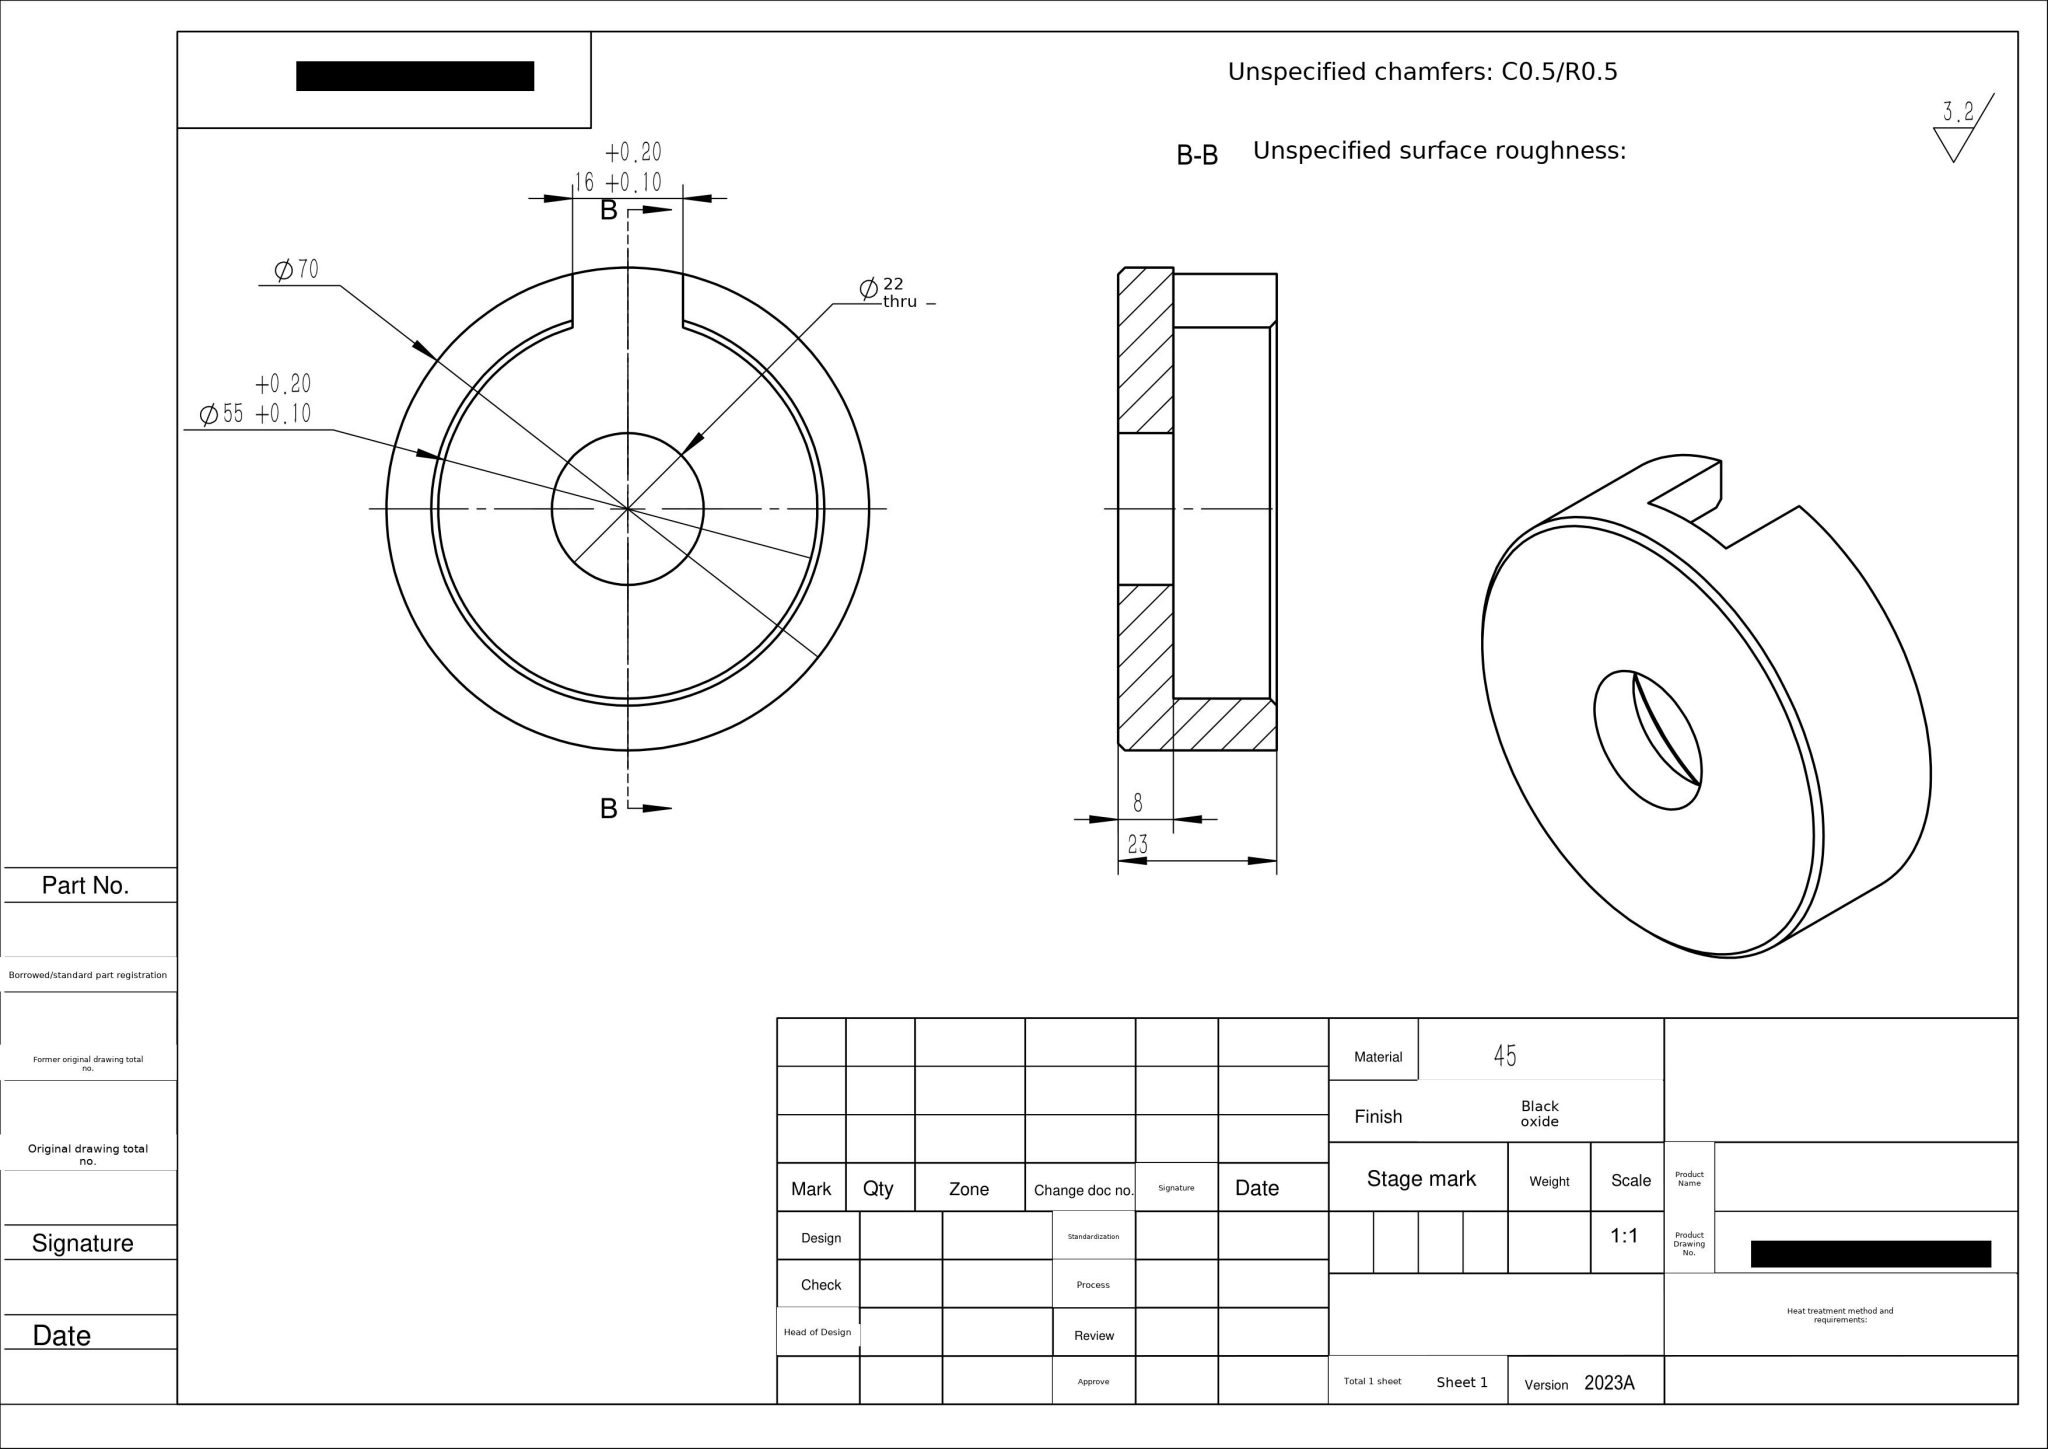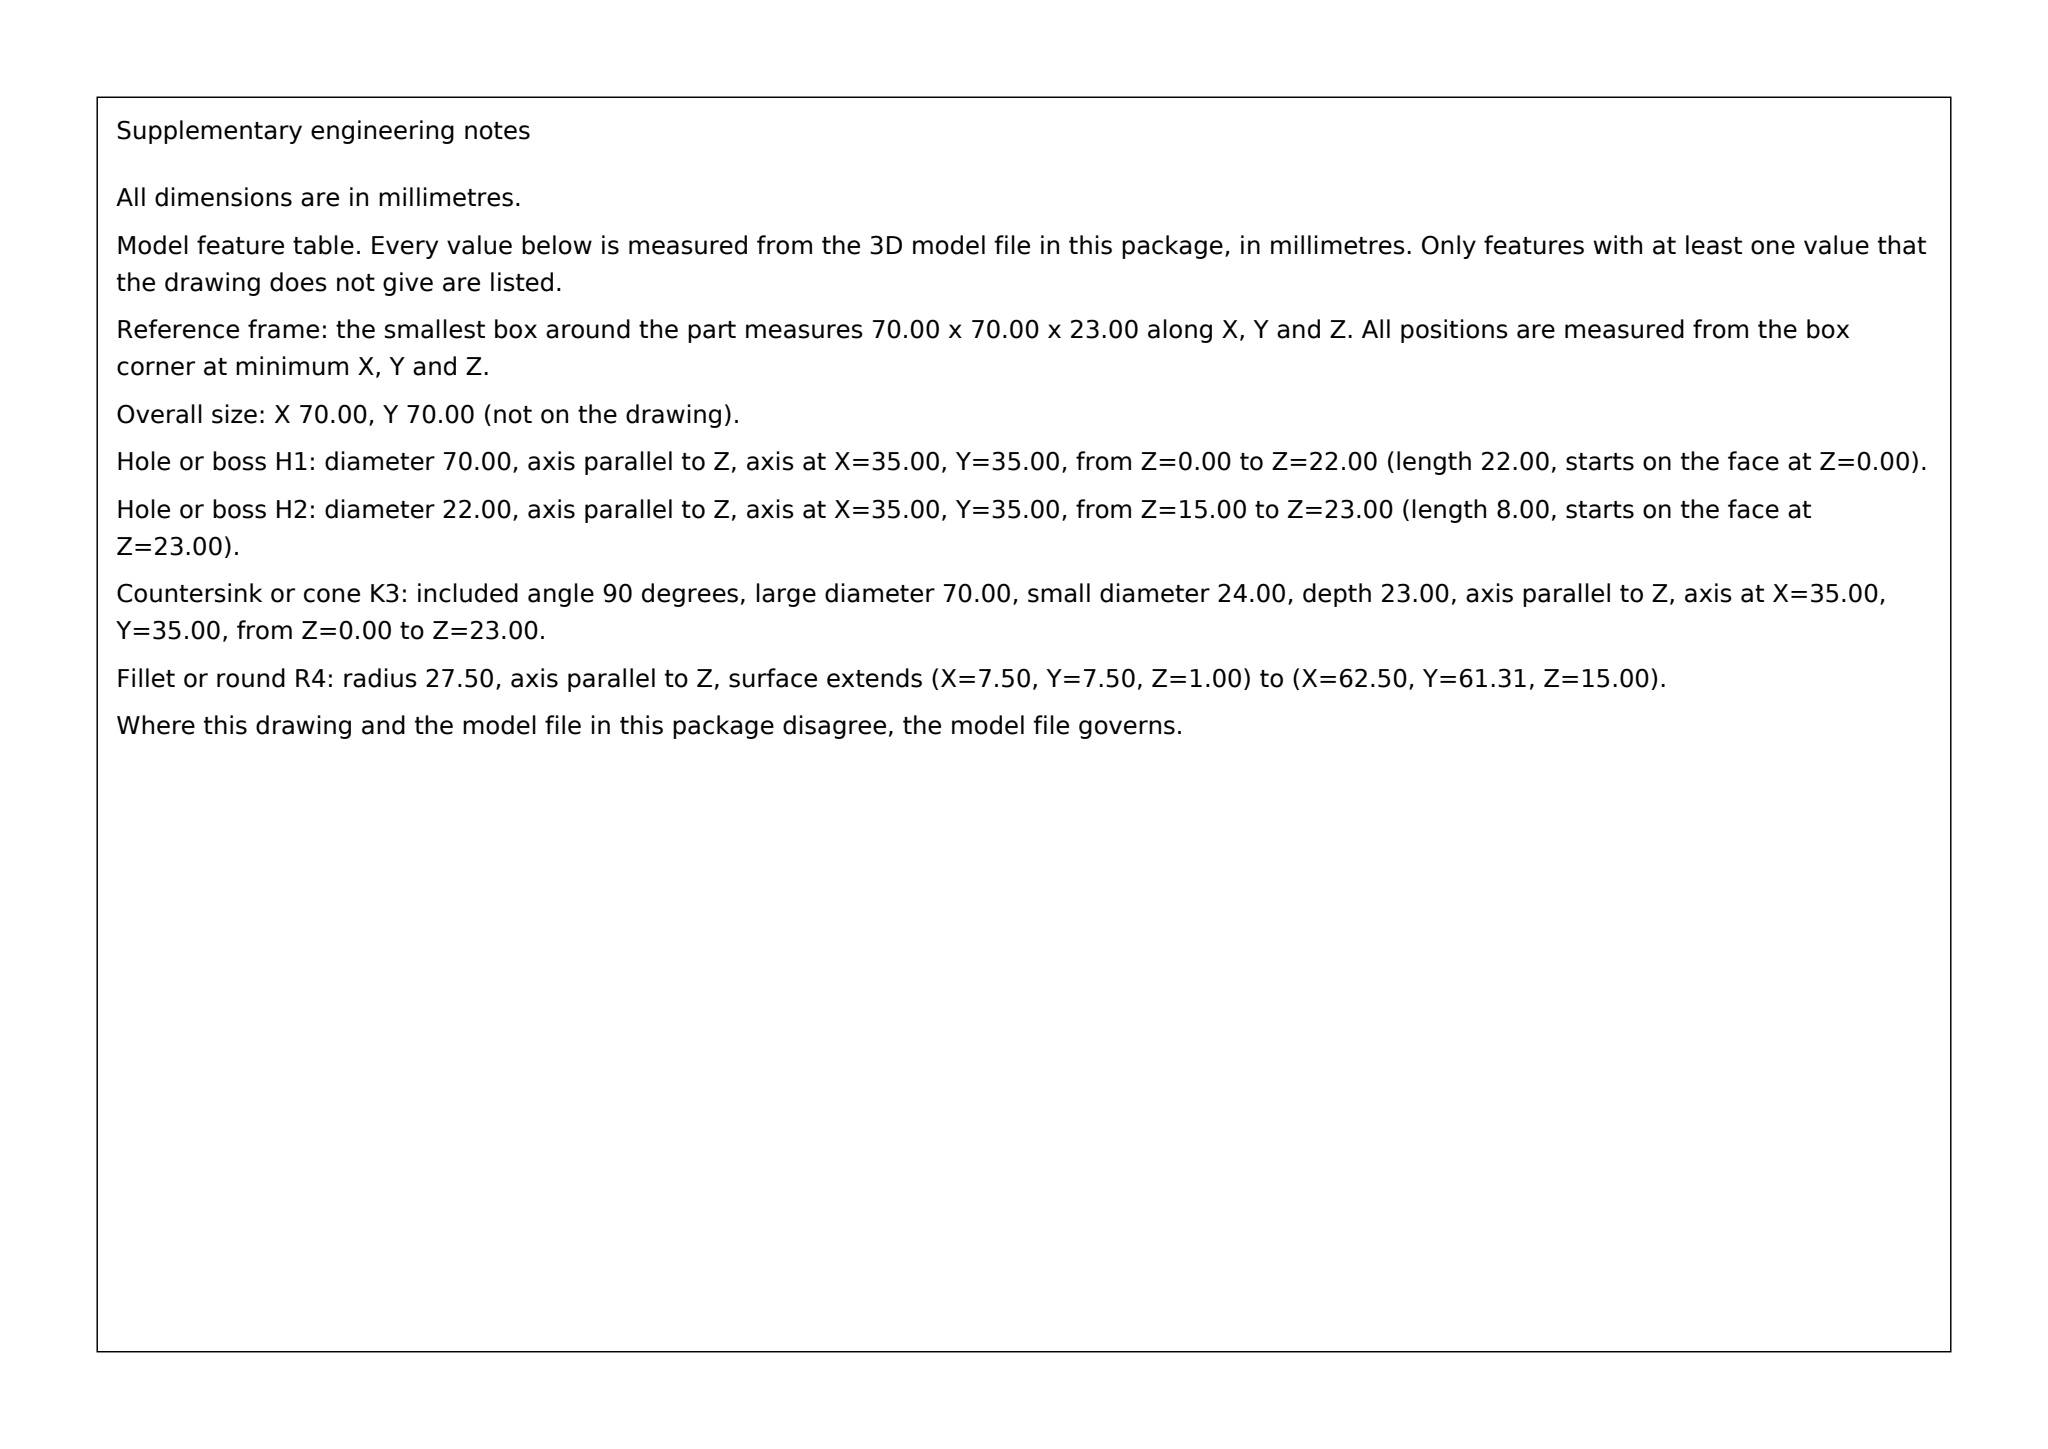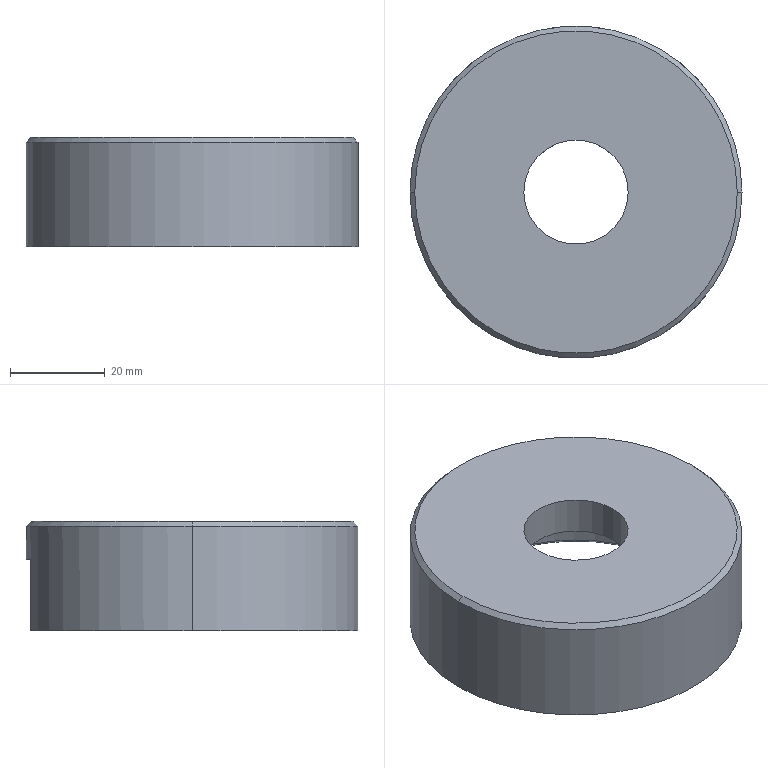Part | SolidWorks | mm | material 45 | 1 solid | 17 faces | box 70 x 70 x 23 mm | volume 47827 mm3 | cylinder 7 | cone 5 | plane 5 | commonest cylinder face diameters 55 x3 70 x2 22 x2
build123d program:
from build123d import *

# Parameters (mm, degrees)
SKETCH1_R           = 35
SKETCH1_R_2         = 11
BOSS_EXTRUDE1_DEPTH = 23
SKETCH2_R           = 27.5
CUT_EXTRUDE1_DEPTH  = 15
SKETCH3_W           = 16
SKETCH3_H           = 43.698
CUT_EXTRUDE2_DEPTH  = 15
CHAMFER1_SIZE       = 1


with BuildPart() as part:
    # Sketch1 → Boss-Extrude1 (new body)
    with BuildSketch(Plane.XY):
        Circle(SKETCH1_R)
        Circle(SKETCH1_R_2, mode=Mode.SUBTRACT)
    extrude(amount=BOSS_EXTRUDE1_DEPTH)

    # Sketch2 → Cut-Extrude1 (cut)
    with BuildSketch(Plane(origin=(0, 0, 0), x_dir=(-1, 0, 0), z_dir=(0, 0, -1))):
        Circle(SKETCH2_R)
    extrude(amount=-CUT_EXTRUDE1_DEPTH, mode=Mode.SUBTRACT)

    # Sketch3 → Cut-Extrude2 (cut)
    with BuildSketch(Plane(origin=(0, 0, 0), x_dir=(-1, 0, 0), z_dir=(0, 0, -1))):
        with Locations((0, 18.087)):
            Rectangle(SKETCH3_W, SKETCH3_H)
    extrude(amount=-CUT_EXTRUDE2_DEPTH, mode=Mode.SUBTRACT)

    # Chamfer1
    chamfer1_edges = [part.edges().sort_by_distance(p)[0] for p in [
        (0, -27.5, 0),
        (-35, 0, 23),
    ]]
    chamfer(chamfer1_edges, length=CHAMFER1_SIZE)


solid = part.part
STEP:
#1=CARTESIAN_POINT('',(34.,0.,23.));
#2=VERTEX_POINT('',#1);
#3=CARTESIAN_POINT('',(-34.,0.,23.));
#4=VERTEX_POINT('',#3);
#5=CARTESIAN_POINT('',(0.,0.,23.));
#6=DIRECTION('',(0.,0.,1.));
#7=DIRECTION('',(1.,0.,0.));
#8=AXIS2_PLACEMENT_3D('',#5,#6,#7);
#9=CIRCLE('',#8,34.);
#10=EDGE_CURVE('',#2,#4,#9,.T.);
#11=ORIENTED_EDGE('',*,*,#10,.F.);
#12=CARTESIAN_POINT('',(35.,0.,22.));
#13=VERTEX_POINT('',#12);
#14=CARTESIAN_POINT('',(34.,0.,23.));
#15=DIRECTION('',(0.7071,0.,-0.7071));
#16=VECTOR('',#15,1000.);
#17=LINE('',#14,#16);
#18=EDGE_CURVE('',#2,#13,#17,.T.);
#19=ORIENTED_EDGE('',*,*,#18,.T.);
#20=CARTESIAN_POINT('',(-35.,0.,22.));
#21=VERTEX_POINT('',#20);
#22=CARTESIAN_POINT('',(0.,0.,22.));
#23=DIRECTION('',(0.,0.,-1.));
#24=DIRECTION('',(1.,0.,0.));
#25=AXIS2_PLACEMENT_3D('',#22,#23,#24);
#26=CIRCLE('',#25,35.);
#27=EDGE_CURVE('',#21,#13,#26,.T.);
#28=ORIENTED_EDGE('',*,*,#27,.F.);
#29=CARTESIAN_POINT('',(-34.,0.,23.));
#30=DIRECTION('',(-0.7071,0.,-0.7071));
#31=VECTOR('',#30,1000.);
#32=LINE('',#29,#31);
#33=EDGE_CURVE('',#4,#21,#32,.T.);
#34=ORIENTED_EDGE('',*,*,#33,.F.);
#35=EDGE_LOOP('',(#11,#19,#28,#34));
#36=FACE_OUTER_BOUND('',#35,.T.);
#37=CARTESIAN_POINT('',(0.,0.,23.));
#38=DIRECTION('',(0.,0.,-1.));
#39=DIRECTION('',(-1.,0.,0.));
#40=AXIS2_PLACEMENT_3D('',#37,#38,#39);
#41=CONICAL_SURFACE('',#40,34.,0.7854);
#42=ADVANCED_FACE('',(#36),#41,.T.);
#43=CARTESIAN_POINT('',(27.5,0.,1.));
#44=VERTEX_POINT('',#43);
#45=CARTESIAN_POINT('',(-27.5,0.,1.));
#46=VERTEX_POINT('',#45);
#47=CARTESIAN_POINT('',(0.,0.,1.));
#48=DIRECTION('',(0.,0.,-1.));
#49=DIRECTION('',(1.,0.,0.));
#50=AXIS2_PLACEMENT_3D('',#47,#48,#49);
#51=CIRCLE('',#50,27.5);
#52=EDGE_CURVE('',#44,#46,#51,.T.);
#53=ORIENTED_EDGE('',*,*,#52,.F.);
#54=CARTESIAN_POINT('',(28.5,0.,0.));
#55=VERTEX_POINT('',#54);
#56=CARTESIAN_POINT('',(27.5,0.,1.));
#57=DIRECTION('',(0.7071,0.,-0.7071));
#58=VECTOR('',#57,1000.);
#59=LINE('',#56,#58);
#60=EDGE_CURVE('',#44,#55,#59,.T.);
#61=ORIENTED_EDGE('',*,*,#60,.T.);
#62=CARTESIAN_POINT('',(-28.5,0.,0.));
#63=VERTEX_POINT('',#62);
#64=CARTESIAN_POINT('',(0.,0.,0.));
#65=DIRECTION('',(0.,0.,1.));
#66=DIRECTION('',(1.,0.,0.));
#67=AXIS2_PLACEMENT_3D('',#64,#65,#66);
#68=CIRCLE('',#67,28.5);
#69=EDGE_CURVE('',#63,#55,#68,.T.);
#70=ORIENTED_EDGE('',*,*,#69,.F.);
#71=CARTESIAN_POINT('',(-27.5,0.,1.));
#72=DIRECTION('',(-0.7071,0.,-0.7071));
#73=VECTOR('',#72,1000.);
#74=LINE('',#71,#73);
#75=EDGE_CURVE('',#46,#63,#74,.T.);
#76=ORIENTED_EDGE('',*,*,#75,.F.);
#77=EDGE_LOOP('',(#53,#61,#70,#76));
#78=FACE_OUTER_BOUND('',#77,.T.);
#79=CARTESIAN_POINT('',(0.,0.,1.));
#80=DIRECTION('',(0.,0.,-1.));
#81=DIRECTION('',(-1.,0.,0.));
#82=AXIS2_PLACEMENT_3D('',#79,#80,#81);
#83=CONICAL_SURFACE('',#82,27.5,0.7854);
#84=ADVANCED_FACE('',(#78),#83,.F.);
#85=CARTESIAN_POINT('',(-8.,26.311,1.));
#86=VERTEX_POINT('',#85);
#87=CARTESIAN_POINT('',(0.,0.,1.));
#88=DIRECTION('',(0.,0.,-1.));
#89=DIRECTION('',(1.,0.,0.));
#90=AXIS2_PLACEMENT_3D('',#87,#88,#89);
#91=CIRCLE('',#90,27.5);
#92=EDGE_CURVE('',#46,#86,#91,.T.);
#93=ORIENTED_EDGE('',*,*,#92,.F.);
#94=ORIENTED_EDGE('',*,*,#75,.T.);
#95=CARTESIAN_POINT('',(-8.,27.354,0.));
#96=VERTEX_POINT('',#95);
#97=CARTESIAN_POINT('',(0.,0.,0.));
#98=DIRECTION('',(0.,0.,1.));
#99=DIRECTION('',(1.,0.,0.));
#100=AXIS2_PLACEMENT_3D('',#97,#98,#99);
#101=CIRCLE('',#100,28.5);
#102=EDGE_CURVE('',#96,#63,#101,.T.);
#103=ORIENTED_EDGE('',*,*,#102,.F.);
#104=CARTESIAN_POINT('',(-8.,26.311,1.));
#105=CARTESIAN_POINT('',(-8.,26.659,0.6669));
#106=CARTESIAN_POINT('',(-8.,27.007,0.3336));
#107=CARTESIAN_POINT('',(-8.,27.354,0.));
#108=B_SPLINE_CURVE_WITH_KNOTS('',3,(#104,#105,#106,#107),.UNSPECIFIED.,.F.,.F.,(4,4),(0.,0.001445),.UNSPECIFIED.);
#109=EDGE_CURVE('',#86,#96,#108,.T.);
#110=ORIENTED_EDGE('',*,*,#109,.F.);
#111=EDGE_LOOP('',(#93,#94,#103,#110));
#112=FACE_OUTER_BOUND('',#111,.T.);
#113=CARTESIAN_POINT('',(0.,0.,1.));
#114=DIRECTION('',(0.,0.,-1.));
#115=DIRECTION('',(-1.,0.,0.));
#116=AXIS2_PLACEMENT_3D('',#113,#114,#115);
#117=CONICAL_SURFACE('',#116,27.5,0.7854);
#118=ADVANCED_FACE('',(#112),#117,.F.);
#119=CARTESIAN_POINT('',(27.5,0.,15.));
#120=VERTEX_POINT('',#119);
#121=CARTESIAN_POINT('',(-27.5,0.,15.));
#122=VERTEX_POINT('',#121);
#123=CARTESIAN_POINT('',(0.,0.,15.));
#124=DIRECTION('',(0.,0.,-1.));
#125=DIRECTION('',(-1.,0.,0.));
#126=AXIS2_PLACEMENT_3D('',#123,#124,#125);
#127=CIRCLE('',#126,27.5);
#128=EDGE_CURVE('',#120,#122,#127,.T.);
#129=ORIENTED_EDGE('',*,*,#128,.F.);
#130=CARTESIAN_POINT('',(27.5,0.,15.));
#131=DIRECTION('',(0.,0.,-1.));
#132=VECTOR('',#131,1000.);
#133=LINE('',#130,#132);
#134=EDGE_CURVE('',#120,#44,#133,.T.);
#135=ORIENTED_EDGE('',*,*,#134,.T.);
#136=ORIENTED_EDGE('',*,*,#52,.T.);
#137=CARTESIAN_POINT('',(-27.5,0.,15.));
#138=DIRECTION('',(0.,0.,-1.));
#139=VECTOR('',#138,1000.);
#140=LINE('',#137,#139);
#141=EDGE_CURVE('',#122,#46,#140,.T.);
#142=ORIENTED_EDGE('',*,*,#141,.F.);
#143=EDGE_LOOP('',(#129,#135,#136,#142));
#144=FACE_OUTER_BOUND('',#143,.T.);
#145=CARTESIAN_POINT('',(0.,0.,15.));
#146=DIRECTION('',(0.,0.,-1.));
#147=DIRECTION('',(-1.,0.,0.));
#148=AXIS2_PLACEMENT_3D('',#145,#146,#147);
#149=CYLINDRICAL_SURFACE('',#148,27.5);
#150=ADVANCED_FACE('',(#144),#149,.F.);
#151=CARTESIAN_POINT('',(-8.,26.311,15.));
#152=VERTEX_POINT('',#151);
#153=CARTESIAN_POINT('',(0.,0.,15.));
#154=DIRECTION('',(0.,0.,-1.));
#155=DIRECTION('',(-1.,0.,0.));
#156=AXIS2_PLACEMENT_3D('',#153,#154,#155);
#157=CIRCLE('',#156,27.5);
#158=EDGE_CURVE('',#122,#152,#157,.T.);
#159=ORIENTED_EDGE('',*,*,#158,.F.);
#160=ORIENTED_EDGE('',*,*,#141,.T.);
#161=ORIENTED_EDGE('',*,*,#92,.T.);
#162=CARTESIAN_POINT('',(-8.,26.311,15.));
#163=DIRECTION('',(0.,0.,1.));
#164=VECTOR('',#163,1000.);
#165=LINE('',#162,#164);
#166=EDGE_CURVE('',#86,#152,#165,.T.);
#167=ORIENTED_EDGE('',*,*,#166,.T.);
#168=EDGE_LOOP('',(#159,#160,#161,#167));
#169=FACE_OUTER_BOUND('',#168,.T.);
#170=CARTESIAN_POINT('',(0.,0.,15.));
#171=DIRECTION('',(0.,0.,-1.));
#172=DIRECTION('',(-1.,0.,0.));
#173=AXIS2_PLACEMENT_3D('',#170,#171,#172);
#174=CYLINDRICAL_SURFACE('',#173,27.5);
#175=ADVANCED_FACE('',(#169),#174,.F.);
#176=ORIENTED_EDGE('',*,*,#27,.T.);
#177=CARTESIAN_POINT('',(35.,0.,0.));
#178=VERTEX_POINT('',#177);
#179=CARTESIAN_POINT('',(35.,0.,23.));
#180=DIRECTION('',(0.,0.,-1.));
#181=VECTOR('',#180,1000.);
#182=LINE('',#179,#181);
#183=EDGE_CURVE('',#13,#178,#182,.T.);
#184=ORIENTED_EDGE('',*,*,#183,.T.);
#185=CARTESIAN_POINT('',(8.,34.073,0.));
#186=VERTEX_POINT('',#185);
#187=CARTESIAN_POINT('',(0.,0.,0.));
#188=DIRECTION('',(0.,0.,1.));
#189=DIRECTION('',(1.,0.,0.));
#190=AXIS2_PLACEMENT_3D('',#187,#188,#189);
#191=CIRCLE('',#190,35.);
#192=EDGE_CURVE('',#178,#186,#191,.T.);
#193=ORIENTED_EDGE('',*,*,#192,.T.);
#194=CARTESIAN_POINT('',(8.,34.073,15.));
#195=VERTEX_POINT('',#194);
#196=CARTESIAN_POINT('',(8.,34.073,23.));
#197=DIRECTION('',(0.,0.,1.));
#198=VECTOR('',#197,1000.);
#199=LINE('',#196,#198);
#200=EDGE_CURVE('',#186,#195,#199,.T.);
#201=ORIENTED_EDGE('',*,*,#200,.T.);
#202=CARTESIAN_POINT('',(-8.,34.073,15.));
#203=VERTEX_POINT('',#202);
#204=CARTESIAN_POINT('',(0.,0.,15.));
#205=DIRECTION('',(0.,0.,-1.));
#206=DIRECTION('',(-1.,0.,0.));
#207=AXIS2_PLACEMENT_3D('',#204,#205,#206);
#208=CIRCLE('',#207,35.);
#209=EDGE_CURVE('',#203,#195,#208,.T.);
#210=ORIENTED_EDGE('',*,*,#209,.F.);
#211=CARTESIAN_POINT('',(-8.,34.073,0.));
#212=VERTEX_POINT('',#211);
#213=CARTESIAN_POINT('',(-8.,34.073,23.));
#214=DIRECTION('',(0.,0.,-1.));
#215=VECTOR('',#214,1000.);
#216=LINE('',#213,#215);
#217=EDGE_CURVE('',#203,#212,#216,.T.);
#218=ORIENTED_EDGE('',*,*,#217,.T.);
#219=CARTESIAN_POINT('',(-35.,0.,0.));
#220=VERTEX_POINT('',#219);
#221=CARTESIAN_POINT('',(0.,0.,0.));
#222=DIRECTION('',(0.,0.,1.));
#223=DIRECTION('',(1.,0.,0.));
#224=AXIS2_PLACEMENT_3D('',#221,#222,#223);
#225=CIRCLE('',#224,35.);
#226=EDGE_CURVE('',#212,#220,#225,.T.);
#227=ORIENTED_EDGE('',*,*,#226,.T.);
#228=CARTESIAN_POINT('',(-35.,0.,23.));
#229=DIRECTION('',(0.,0.,-1.));
#230=VECTOR('',#229,1000.);
#231=LINE('',#228,#230);
#232=EDGE_CURVE('',#21,#220,#231,.T.);
#233=ORIENTED_EDGE('',*,*,#232,.F.);
#234=EDGE_LOOP('',(#176,#184,#193,#201,#210,#218,#227,#233));
#235=FACE_OUTER_BOUND('',#234,.T.);
#236=CARTESIAN_POINT('',(0.,0.,23.));
#237=DIRECTION('',(0.,0.,-1.));
#238=DIRECTION('',(-1.,0.,0.));
#239=AXIS2_PLACEMENT_3D('',#236,#237,#238);
#240=CYLINDRICAL_SURFACE('',#239,35.);
#241=ADVANCED_FACE('',(#235),#240,.T.);
#242=CARTESIAN_POINT('',(-11.,0.,23.));
#243=VERTEX_POINT('',#242);
#244=CARTESIAN_POINT('',(11.,0.,23.));
#245=VERTEX_POINT('',#244);
#246=CARTESIAN_POINT('',(0.,0.,23.));
#247=DIRECTION('',(0.,0.,1.));
#248=DIRECTION('',(1.,0.,0.));
#249=AXIS2_PLACEMENT_3D('',#246,#247,#248);
#250=CIRCLE('',#249,11.);
#251=EDGE_CURVE('',#243,#245,#250,.T.);
#252=ORIENTED_EDGE('',*,*,#251,.T.);
#253=CARTESIAN_POINT('',(11.,0.,15.));
#254=VERTEX_POINT('',#253);
#255=CARTESIAN_POINT('',(11.,0.,23.));
#256=DIRECTION('',(0.,0.,-1.));
#257=VECTOR('',#256,1000.);
#258=LINE('',#255,#257);
#259=EDGE_CURVE('',#245,#254,#258,.T.);
#260=ORIENTED_EDGE('',*,*,#259,.T.);
#261=CARTESIAN_POINT('',(-11.,0.,15.));
#262=VERTEX_POINT('',#261);
#263=CARTESIAN_POINT('',(0.,0.,15.));
#264=DIRECTION('',(0.,0.,-1.));
#265=DIRECTION('',(-1.,0.,0.));
#266=AXIS2_PLACEMENT_3D('',#263,#264,#265);
#267=CIRCLE('',#266,11.);
#268=EDGE_CURVE('',#254,#262,#267,.T.);
#269=ORIENTED_EDGE('',*,*,#268,.T.);
#270=CARTESIAN_POINT('',(-11.,0.,23.));
#271=DIRECTION('',(0.,0.,-1.));
#272=VECTOR('',#271,1000.);
#273=LINE('',#270,#272);
#274=EDGE_CURVE('',#243,#262,#273,.T.);
#275=ORIENTED_EDGE('',*,*,#274,.F.);
#276=EDGE_LOOP('',(#252,#260,#269,#275));
#277=FACE_OUTER_BOUND('',#276,.T.);
#278=CARTESIAN_POINT('',(0.,0.,23.));
#279=DIRECTION('',(0.,0.,-1.));
#280=DIRECTION('',(-1.,0.,0.));
#281=AXIS2_PLACEMENT_3D('',#278,#279,#280);
#282=CYLINDRICAL_SURFACE('',#281,11.);
#283=ADVANCED_FACE('',(#277),#282,.F.);
#284=ORIENTED_EDGE('',*,*,#259,.F.);
#285=CARTESIAN_POINT('',(0.,0.,23.));
#286=DIRECTION('',(0.,0.,1.));
#287=DIRECTION('',(1.,0.,0.));
#288=AXIS2_PLACEMENT_3D('',#285,#286,#287);
#289=CIRCLE('',#288,11.);
#290=EDGE_CURVE('',#245,#243,#289,.T.);
#291=ORIENTED_EDGE('',*,*,#290,.T.);
#292=ORIENTED_EDGE('',*,*,#274,.T.);
#293=CARTESIAN_POINT('',(0.,0.,15.));
#294=DIRECTION('',(0.,0.,-1.));
#295=DIRECTION('',(-1.,0.,0.));
#296=AXIS2_PLACEMENT_3D('',#293,#294,#295);
#297=CIRCLE('',#296,11.);
#298=EDGE_CURVE('',#262,#254,#297,.T.);
#299=ORIENTED_EDGE('',*,*,#298,.T.);
#300=EDGE_LOOP('',(#284,#291,#292,#299));
#301=FACE_OUTER_BOUND('',#300,.T.);
#302=CARTESIAN_POINT('',(0.,0.,23.));
#303=DIRECTION('',(0.,0.,-1.));
#304=DIRECTION('',(-1.,0.,0.));
#305=AXIS2_PLACEMENT_3D('',#302,#303,#304);
#306=CYLINDRICAL_SURFACE('',#305,11.);
#307=ADVANCED_FACE('',(#301),#306,.F.);
#308=CARTESIAN_POINT('',(0.,0.,23.));
#309=DIRECTION('',(0.,0.,1.));
#310=DIRECTION('',(1.,0.,0.));
#311=AXIS2_PLACEMENT_3D('',#308,#309,#310);
#312=CIRCLE('',#311,34.);
#313=EDGE_CURVE('',#4,#2,#312,.T.);
#314=ORIENTED_EDGE('',*,*,#313,.T.);
#315=ORIENTED_EDGE('',*,*,#10,.T.);
#316=EDGE_LOOP('',(#314,#315));
#317=FACE_OUTER_BOUND('',#316,.T.);
#318=ORIENTED_EDGE('',*,*,#251,.F.);
#319=ORIENTED_EDGE('',*,*,#290,.F.);
#320=EDGE_LOOP('',(#318,#319));
#321=FACE_BOUND('',#320,.T.);
#322=CARTESIAN_POINT('',(0.,0.,23.));
#323=DIRECTION('',(0.,0.,1.));
#324=DIRECTION('',(1.,0.,0.));
#325=AXIS2_PLACEMENT_3D('',#322,#323,#324);
#326=PLANE('',#325);
#327=ADVANCED_FACE('',(#317,#321),#326,.T.);
#328=CARTESIAN_POINT('',(-8.,-3.762,0.));
#329=DIRECTION('',(0.,1.,0.));
#330=VECTOR('',#329,1000.);
#331=LINE('',#328,#330);
#332=EDGE_CURVE('',#96,#212,#331,.T.);
#333=ORIENTED_EDGE('',*,*,#332,.F.);
#334=ORIENTED_EDGE('',*,*,#102,.T.);
#335=ORIENTED_EDGE('',*,*,#69,.T.);
#336=CARTESIAN_POINT('',(8.,27.354,0.));
#337=VERTEX_POINT('',#336);
#338=CARTESIAN_POINT('',(0.,0.,0.));
#339=DIRECTION('',(0.,0.,1.));
#340=DIRECTION('',(1.,0.,0.));
#341=AXIS2_PLACEMENT_3D('',#338,#339,#340);
#342=CIRCLE('',#341,28.5);
#343=EDGE_CURVE('',#55,#337,#342,.T.);
#344=ORIENTED_EDGE('',*,*,#343,.T.);
#345=CARTESIAN_POINT('',(8.,-3.762,0.));
#346=DIRECTION('',(0.,-1.,0.));
#347=VECTOR('',#346,1000.);
#348=LINE('',#345,#347);
#349=EDGE_CURVE('',#186,#337,#348,.T.);
#350=ORIENTED_EDGE('',*,*,#349,.F.);
#351=ORIENTED_EDGE('',*,*,#192,.F.);
#352=CARTESIAN_POINT('',(0.,0.,0.));
#353=DIRECTION('',(0.,0.,1.));
#354=DIRECTION('',(1.,0.,0.));
#355=AXIS2_PLACEMENT_3D('',#352,#353,#354);
#356=CIRCLE('',#355,35.);
#357=EDGE_CURVE('',#220,#178,#356,.T.);
#358=ORIENTED_EDGE('',*,*,#357,.F.);
#359=ORIENTED_EDGE('',*,*,#226,.F.);
#360=EDGE_LOOP('',(#333,#334,#335,#344,#350,#351,#358,#359));
#361=FACE_OUTER_BOUND('',#360,.T.);
#362=CARTESIAN_POINT('',(0.,0.,0.));
#363=DIRECTION('',(0.,0.,1.));
#364=DIRECTION('',(1.,0.,0.));
#365=AXIS2_PLACEMENT_3D('',#362,#363,#364);
#366=PLANE('',#365);
#367=ADVANCED_FACE('',(#361),#366,.F.);
#368=ORIENTED_EDGE('',*,*,#183,.F.);
#369=CARTESIAN_POINT('',(0.,0.,22.));
#370=DIRECTION('',(0.,0.,-1.));
#371=DIRECTION('',(1.,0.,0.));
#372=AXIS2_PLACEMENT_3D('',#369,#370,#371);
#373=CIRCLE('',#372,35.);
#374=EDGE_CURVE('',#13,#21,#373,.T.);
#375=ORIENTED_EDGE('',*,*,#374,.T.);
#376=ORIENTED_EDGE('',*,*,#232,.T.);
#377=ORIENTED_EDGE('',*,*,#357,.T.);
#378=EDGE_LOOP('',(#368,#375,#376,#377));
#379=FACE_OUTER_BOUND('',#378,.T.);
#380=CARTESIAN_POINT('',(0.,0.,23.));
#381=DIRECTION('',(0.,0.,-1.));
#382=DIRECTION('',(-1.,0.,0.));
#383=AXIS2_PLACEMENT_3D('',#380,#381,#382);
#384=CYLINDRICAL_SURFACE('',#383,35.);
#385=ADVANCED_FACE('',(#379),#384,.T.);
#386=ORIENTED_EDGE('',*,*,#134,.F.);
#387=CARTESIAN_POINT('',(8.,26.311,15.));
#388=VERTEX_POINT('',#387);
#389=CARTESIAN_POINT('',(0.,0.,15.));
#390=DIRECTION('',(0.,0.,-1.));
#391=DIRECTION('',(-1.,0.,0.));
#392=AXIS2_PLACEMENT_3D('',#389,#390,#391);
#393=CIRCLE('',#392,27.5);
#394=EDGE_CURVE('',#388,#120,#393,.T.);
#395=ORIENTED_EDGE('',*,*,#394,.F.);
#396=CARTESIAN_POINT('',(8.,26.311,1.));
#397=VERTEX_POINT('',#396);
#398=CARTESIAN_POINT('',(8.,26.311,15.));
#399=DIRECTION('',(0.,0.,-1.));
#400=VECTOR('',#399,1000.);
#401=LINE('',#398,#400);
#402=EDGE_CURVE('',#388,#397,#401,.T.);
#403=ORIENTED_EDGE('',*,*,#402,.T.);
#404=CARTESIAN_POINT('',(0.,0.,1.));
#405=DIRECTION('',(0.,0.,-1.));
#406=DIRECTION('',(1.,0.,0.));
#407=AXIS2_PLACEMENT_3D('',#404,#405,#406);
#408=CIRCLE('',#407,27.5);
#409=EDGE_CURVE('',#397,#44,#408,.T.);
#410=ORIENTED_EDGE('',*,*,#409,.T.);
#411=EDGE_LOOP('',(#386,#395,#403,#410));
#412=FACE_OUTER_BOUND('',#411,.T.);
#413=CARTESIAN_POINT('',(0.,0.,15.));
#414=DIRECTION('',(0.,0.,-1.));
#415=DIRECTION('',(-1.,0.,0.));
#416=AXIS2_PLACEMENT_3D('',#413,#414,#415);
#417=CYLINDRICAL_SURFACE('',#416,27.5);
#418=ADVANCED_FACE('',(#412),#417,.F.);
#419=ORIENTED_EDGE('',*,*,#298,.F.);
#420=ORIENTED_EDGE('',*,*,#268,.F.);
#421=EDGE_LOOP('',(#419,#420));
#422=FACE_BOUND('',#421,.T.);
#423=ORIENTED_EDGE('',*,*,#394,.T.);
#424=ORIENTED_EDGE('',*,*,#128,.T.);
#425=ORIENTED_EDGE('',*,*,#158,.T.);
#426=CARTESIAN_POINT('',(-8.,-3.762,15.));
#427=DIRECTION('',(0.,1.,0.));
#428=VECTOR('',#427,1000.);
#429=LINE('',#426,#428);
#430=EDGE_CURVE('',#152,#203,#429,.T.);
#431=ORIENTED_EDGE('',*,*,#430,.T.);
#432=ORIENTED_EDGE('',*,*,#209,.T.);
#433=CARTESIAN_POINT('',(8.,-3.762,15.));
#434=DIRECTION('',(0.,-1.,0.));
#435=VECTOR('',#434,1000.);
#436=LINE('',#433,#435);
#437=EDGE_CURVE('',#195,#388,#436,.T.);
#438=ORIENTED_EDGE('',*,*,#437,.T.);
#439=EDGE_LOOP('',(#423,#424,#425,#431,#432,#438));
#440=FACE_OUTER_BOUND('',#439,.T.);
#441=CARTESIAN_POINT('',(0.,0.,15.));
#442=DIRECTION('',(0.,0.,-1.));
#443=DIRECTION('',(-1.,0.,0.));
#444=AXIS2_PLACEMENT_3D('',#441,#442,#443);
#445=PLANE('',#444);
#446=ADVANCED_FACE('',(#422,#440),#445,.T.);
#447=ORIENTED_EDGE('',*,*,#349,.T.);
#448=CARTESIAN_POINT('',(8.,27.354,0.));
#449=CARTESIAN_POINT('',(8.,27.007,0.3336));
#450=CARTESIAN_POINT('',(8.,26.659,0.6669));
#451=CARTESIAN_POINT('',(8.,26.311,1.));
#452=B_SPLINE_CURVE_WITH_KNOTS('',3,(#448,#449,#450,#451),.UNSPECIFIED.,.F.,.F.,(4,4),(0.,0.001445),.UNSPECIFIED.);
#453=EDGE_CURVE('',#337,#397,#452,.T.);
#454=ORIENTED_EDGE('',*,*,#453,.T.);
#455=ORIENTED_EDGE('',*,*,#402,.F.);
#456=ORIENTED_EDGE('',*,*,#437,.F.);
#457=ORIENTED_EDGE('',*,*,#200,.F.);
#458=EDGE_LOOP('',(#447,#454,#455,#456,#457));
#459=FACE_OUTER_BOUND('',#458,.T.);
#460=CARTESIAN_POINT('',(8.,-3.762,15.));
#461=DIRECTION('',(1.,0.,0.));
#462=DIRECTION('',(0.,0.,-1.));
#463=AXIS2_PLACEMENT_3D('',#460,#461,#462);
#464=PLANE('',#463);
#465=ADVANCED_FACE('',(#459),#464,.F.);
#466=ORIENTED_EDGE('',*,*,#166,.F.);
#467=ORIENTED_EDGE('',*,*,#109,.T.);
#468=ORIENTED_EDGE('',*,*,#332,.T.);
#469=ORIENTED_EDGE('',*,*,#217,.F.);
#470=ORIENTED_EDGE('',*,*,#430,.F.);
#471=EDGE_LOOP('',(#466,#467,#468,#469,#470));
#472=FACE_OUTER_BOUND('',#471,.T.);
#473=CARTESIAN_POINT('',(-8.,-3.762,15.));
#474=DIRECTION('',(-1.,0.,0.));
#475=DIRECTION('',(0.,0.,1.));
#476=AXIS2_PLACEMENT_3D('',#473,#474,#475);
#477=PLANE('',#476);
#478=ADVANCED_FACE('',(#472),#477,.F.);
#479=ORIENTED_EDGE('',*,*,#60,.F.);
#480=ORIENTED_EDGE('',*,*,#409,.F.);
#481=ORIENTED_EDGE('',*,*,#453,.F.);
#482=ORIENTED_EDGE('',*,*,#343,.F.);
#483=EDGE_LOOP('',(#479,#480,#481,#482));
#484=FACE_OUTER_BOUND('',#483,.T.);
#485=CARTESIAN_POINT('',(0.,0.,1.));
#486=DIRECTION('',(0.,0.,-1.));
#487=DIRECTION('',(-1.,0.,0.));
#488=AXIS2_PLACEMENT_3D('',#485,#486,#487);
#489=CONICAL_SURFACE('',#488,27.5,0.7854);
#490=ADVANCED_FACE('',(#484),#489,.F.);
#491=ORIENTED_EDGE('',*,*,#18,.F.);
#492=ORIENTED_EDGE('',*,*,#313,.F.);
#493=ORIENTED_EDGE('',*,*,#33,.T.);
#494=ORIENTED_EDGE('',*,*,#374,.F.);
#495=EDGE_LOOP('',(#491,#492,#493,#494));
#496=FACE_OUTER_BOUND('',#495,.T.);
#497=CARTESIAN_POINT('',(0.,0.,23.));
#498=DIRECTION('',(0.,0.,-1.));
#499=DIRECTION('',(-1.,0.,0.));
#500=AXIS2_PLACEMENT_3D('',#497,#498,#499);
#501=CONICAL_SURFACE('',#500,34.,0.7854);
#502=ADVANCED_FACE('',(#496),#501,.T.);
#503=CLOSED_SHELL('',(#42,#84,#118,#150,#175,#241,#283,#307,#327,#367,#385,#418,#446,#465,#478,#490,#502));
#504=MANIFOLD_SOLID_BREP('',#503);
#505=CARTESIAN_POINT('',(0.,0.,0.));
#506=DIRECTION('',(0.,0.,1.));
#507=DIRECTION('',(1.,0.,0.));
#508=AXIS2_PLACEMENT_3D('',#505,#506,#507);
#509=(LENGTH_UNIT()NAMED_UNIT(*)SI_UNIT(.MILLI.,.METRE.));
#510=UNCERTAINTY_MEASURE_WITH_UNIT(LENGTH_MEASURE(0.00001),#509,'','');
#511=(NAMED_UNIT(*)PLANE_ANGLE_UNIT()SI_UNIT($,.RADIAN.));
#512=(NAMED_UNIT(*)SI_UNIT($,.STERADIAN.)SOLID_ANGLE_UNIT());
#513=(GEOMETRIC_REPRESENTATION_CONTEXT(3)GLOBAL_UNCERTAINTY_ASSIGNED_CONTEXT((#510))GLOBAL_UNIT_ASSIGNED_CONTEXT((#509,#511,#512))REPRESENTATION_CONTEXT('',''));
#514=ADVANCED_BREP_SHAPE_REPRESENTATION('',(#504,#508),#513);